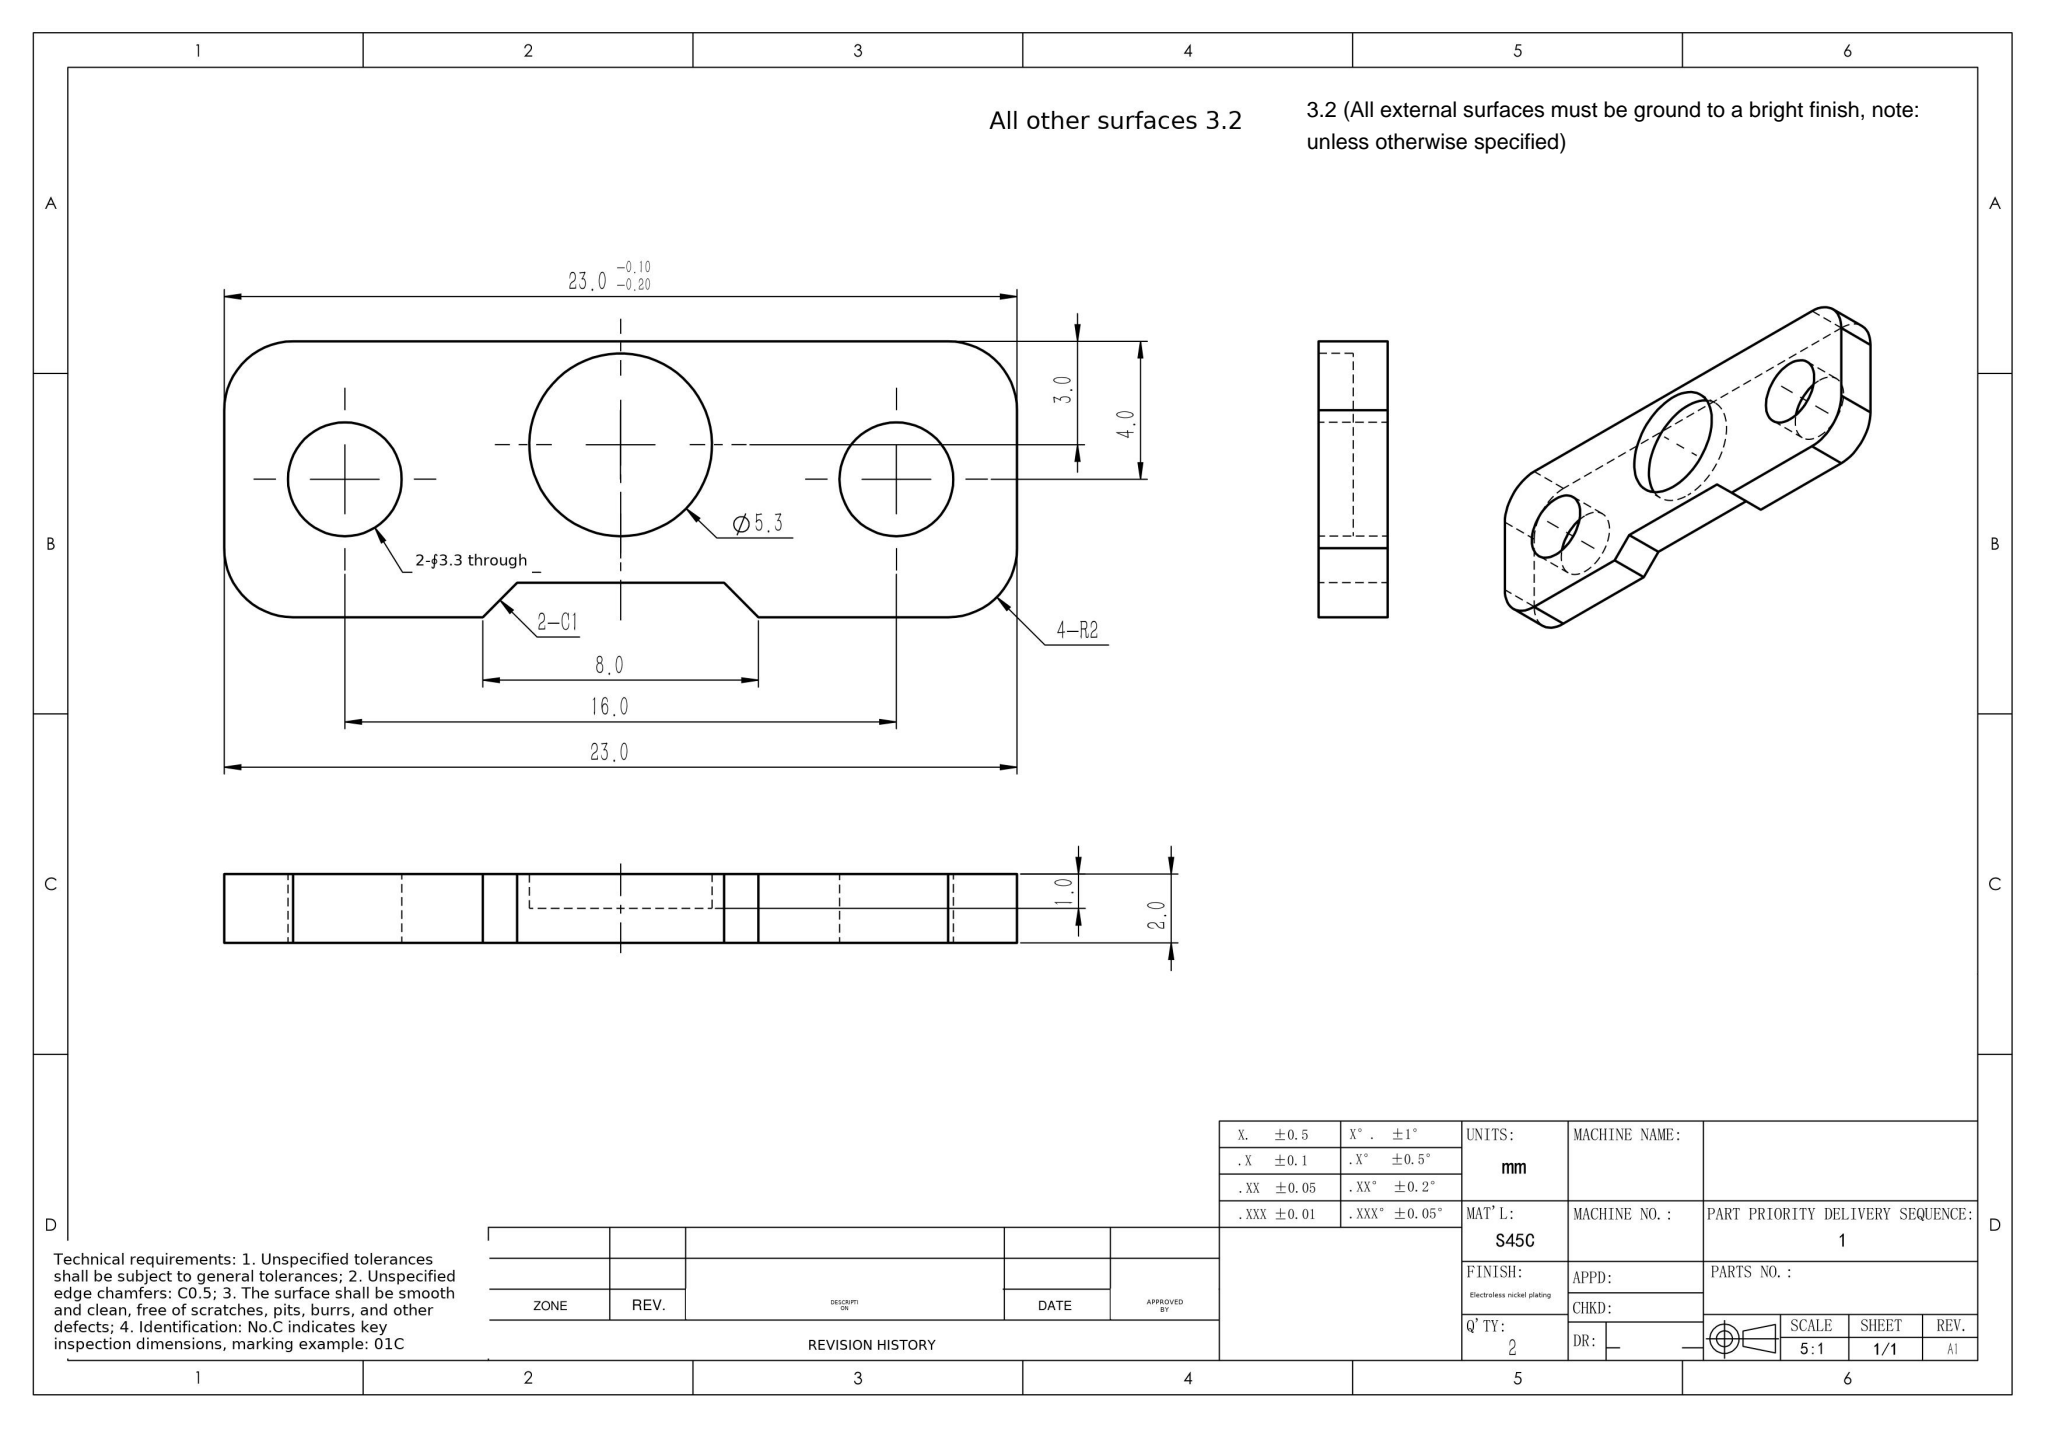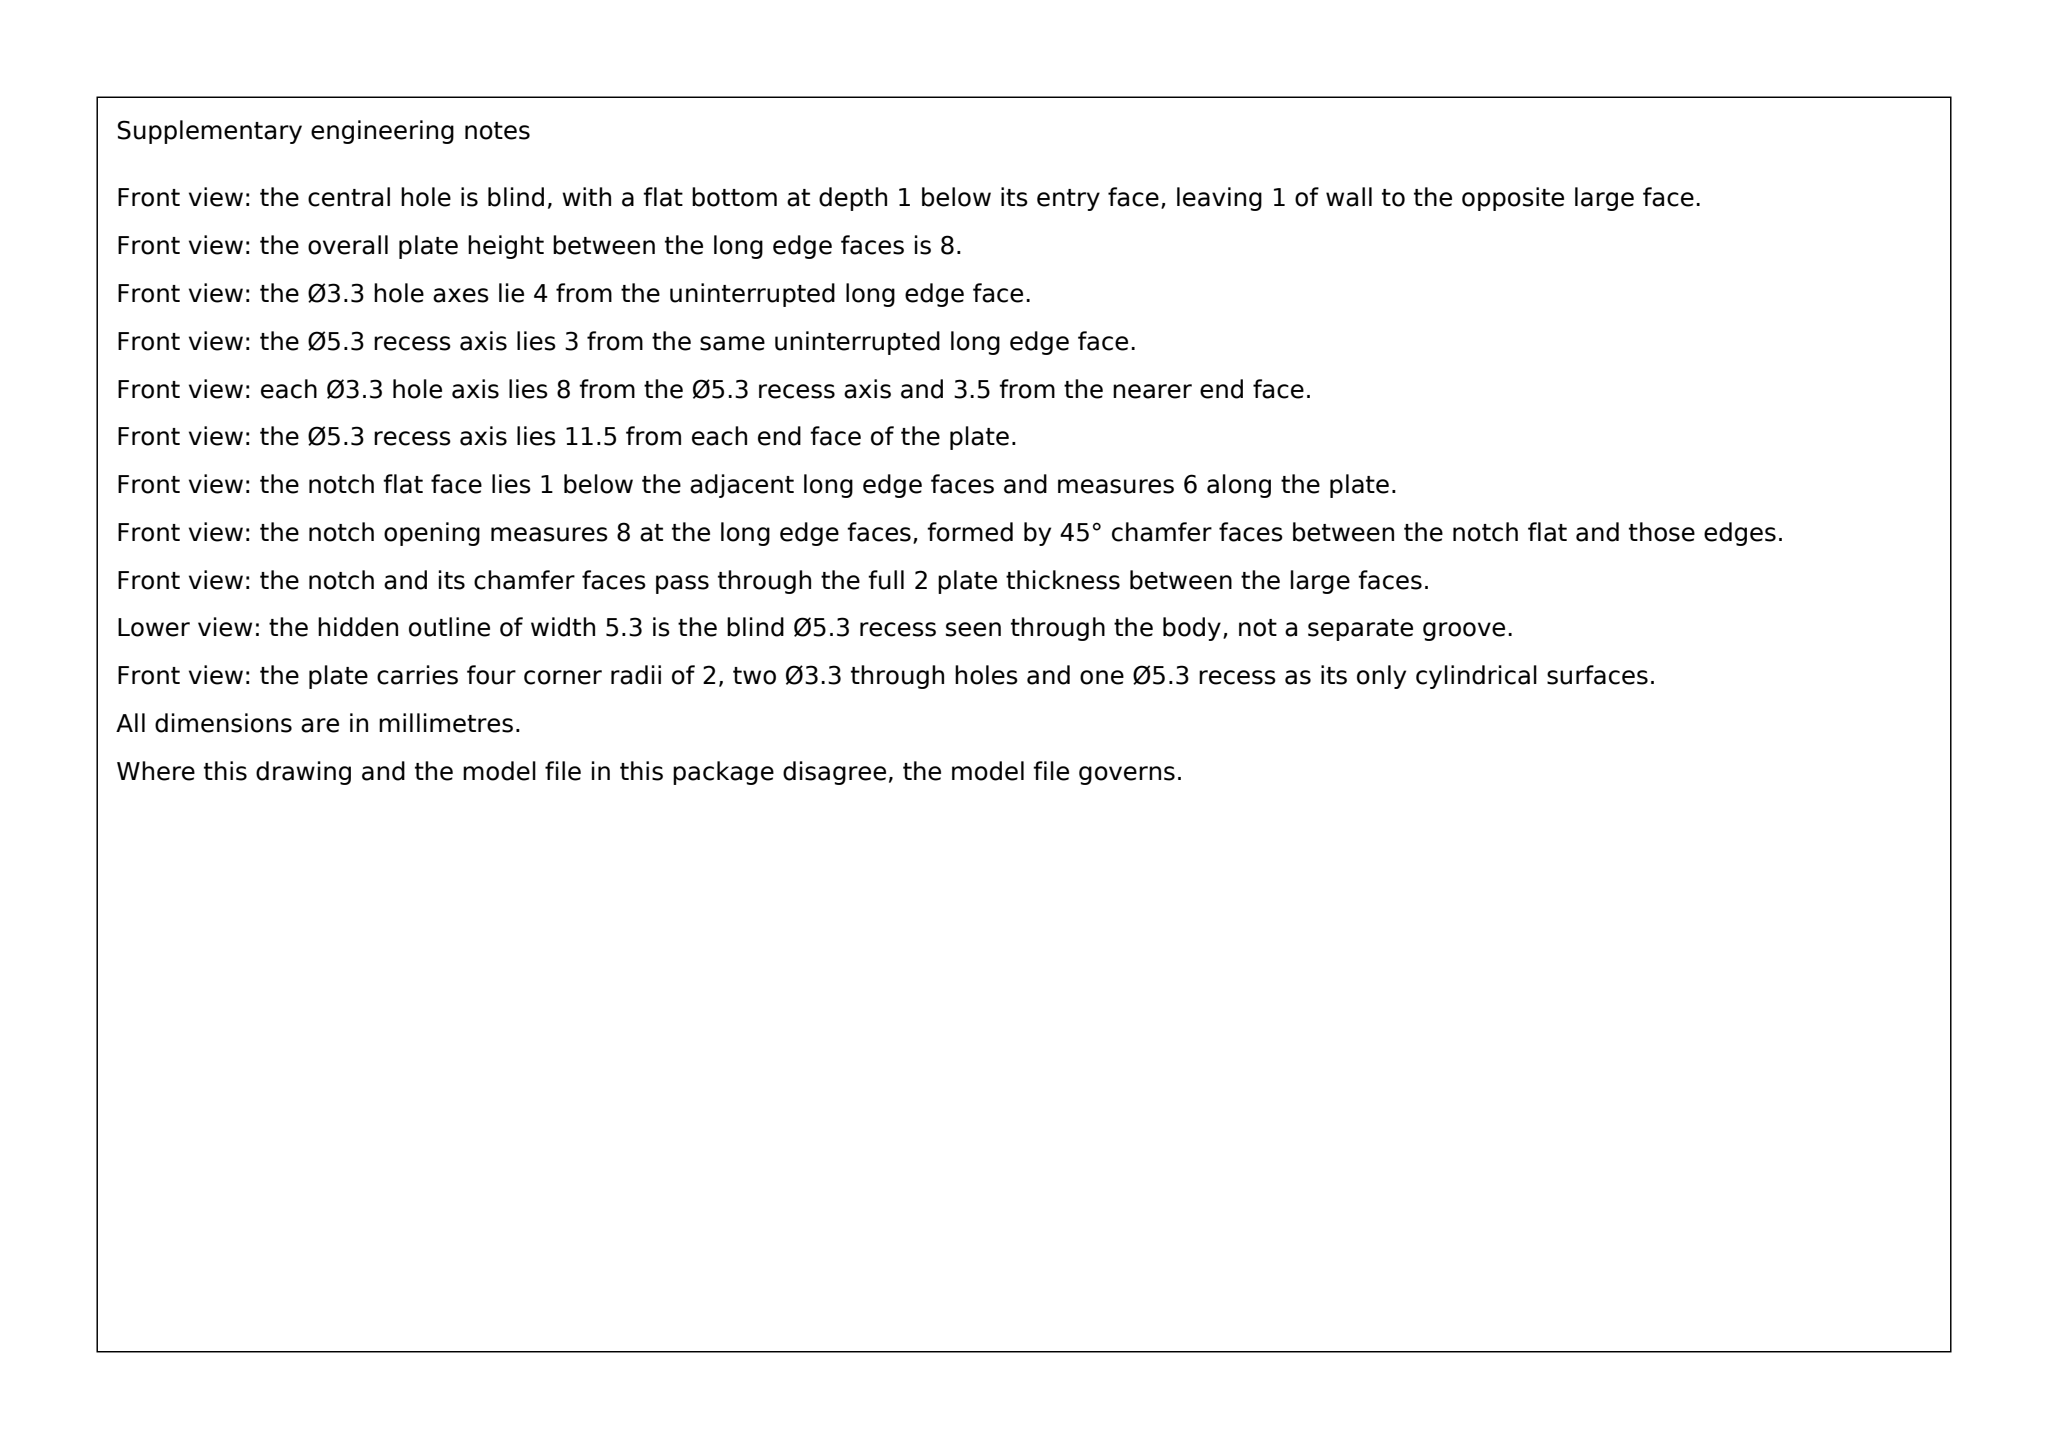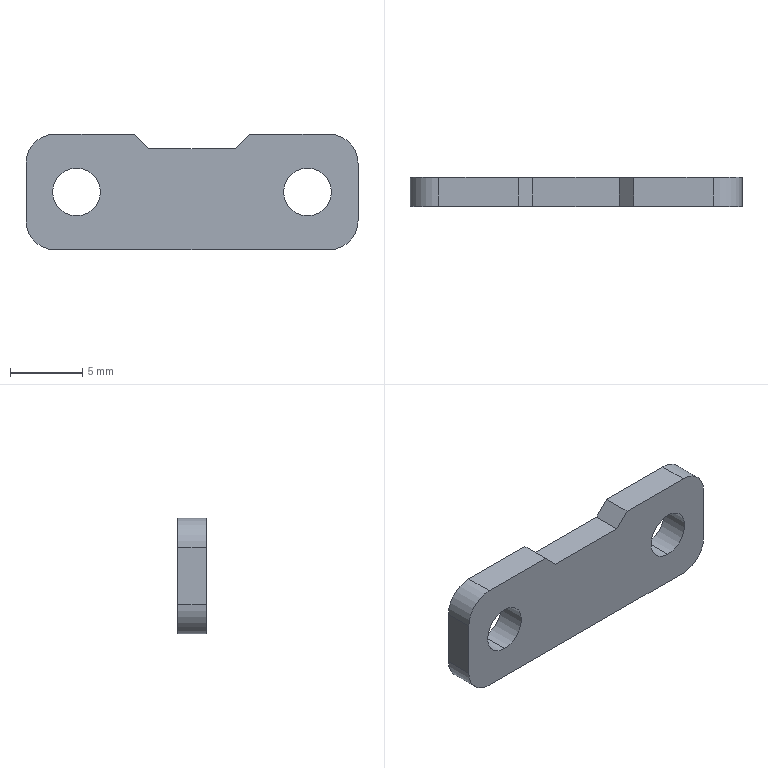Part | SolidWorks | mm | material S45C | 1 solid | 21 faces | box 23 x 2 x 8 mm | volume 291 mm3 | plane 11 | cylinder 10 | commonest cylinder face diameters 3.3 x4 4 x4 5.3 x2
Drawing notes:
Overall height 8.0 from bottom face to top face (plate 23.0 long x 8.0 high x 2.0 thick) | from the solid: bbox_xyz [23.0, 2.0, 8.0]
2X Ø3.3 THRU (2.0 deep), located 3.5 and 19.5 from left end, 4.0 up from bottom edge | from the solid: cylinders dia 3.3, axis y, pos [3.5,null,4.0] and [19.5,null,4.0], length 2.0
Ø5.3 C'BORE 1.0 DEEP both faces, centered 11.5 from left end, 3.0 up from bottom edge | from the solid: cylinders dia 5.3, axis y, pos [11.5,null,3.0], length 1.0, count 2
Overall part width 8.0 across the front view, measured from the back face (Z0 datum). | from the solid: bbox_xyz = [23.0, 2.0, 8.0]
2X Ø3.3 THRU, on hole centerline 4.0 from back face, located 3.5 and 19.5 from left end face (X0 datum). | from the solid: cylinders 3.3 dia, axis y, pos [3.5,null,4.0] and [19.5,null,4.0], length 2.0
Ø5.3 hole, depth 1.0 from each face, center 11.5 from left end face and 3.0 from back face. | from the solid: cylinders 5.3 dia, axis y, pos [11.5,null,3.0], length 1.0, count 2
STEP:
#1=CARTESIAN_POINT('',(8.,2.,-1.65));
#2=VERTEX_POINT('',#1);
#3=CARTESIAN_POINT('',(8.,2.,1.65));
#4=VERTEX_POINT('',#3);
#5=CARTESIAN_POINT('',(8.,2.,0.));
#6=DIRECTION('',(0.,1.,0.));
#7=DIRECTION('',(0.,0.,-1.));
#8=AXIS2_PLACEMENT_3D('',#5,#6,#7);
#9=CIRCLE('',#8,1.65);
#10=EDGE_CURVE('',#2,#4,#9,.T.);
#11=ORIENTED_EDGE('',*,*,#10,.T.);
#12=CARTESIAN_POINT('',(8.,0.,1.65));
#13=VERTEX_POINT('',#12);
#14=CARTESIAN_POINT('',(8.,6.667,1.65));
#15=DIRECTION('',(0.,-1.,0.));
#16=VECTOR('',#15,1000.);
#17=LINE('',#14,#16);
#18=EDGE_CURVE('',#4,#13,#17,.T.);
#19=ORIENTED_EDGE('',*,*,#18,.T.);
#20=CARTESIAN_POINT('',(8.,0.,-1.65));
#21=VERTEX_POINT('',#20);
#22=CARTESIAN_POINT('',(8.,0.,0.));
#23=DIRECTION('',(0.,-1.,0.));
#24=DIRECTION('',(0.,0.,-1.));
#25=AXIS2_PLACEMENT_3D('',#22,#23,#24);
#26=CIRCLE('',#25,1.65);
#27=EDGE_CURVE('',#13,#21,#26,.T.);
#28=ORIENTED_EDGE('',*,*,#27,.T.);
#29=CARTESIAN_POINT('',(8.,6.667,-1.65));
#30=DIRECTION('',(0.,-1.,0.));
#31=VECTOR('',#30,1000.);
#32=LINE('',#29,#31);
#33=EDGE_CURVE('',#2,#21,#32,.T.);
#34=ORIENTED_EDGE('',*,*,#33,.F.);
#35=EDGE_LOOP('',(#11,#19,#28,#34));
#36=FACE_OUTER_BOUND('',#35,.T.);
#37=CARTESIAN_POINT('',(8.,6.667,0.));
#38=DIRECTION('',(0.,-1.,0.));
#39=DIRECTION('',(0.,0.,-1.));
#40=AXIS2_PLACEMENT_3D('',#37,#38,#39);
#41=CYLINDRICAL_SURFACE('',#40,1.65);
#42=ADVANCED_FACE('',(#36),#41,.F.);
#43=CARTESIAN_POINT('',(-8.,2.,-1.65));
#44=VERTEX_POINT('',#43);
#45=CARTESIAN_POINT('',(-8.,2.,1.65));
#46=VERTEX_POINT('',#45);
#47=CARTESIAN_POINT('',(-8.,2.,0.));
#48=DIRECTION('',(0.,1.,0.));
#49=DIRECTION('',(0.,0.,-1.));
#50=AXIS2_PLACEMENT_3D('',#47,#48,#49);
#51=CIRCLE('',#50,1.65);
#52=EDGE_CURVE('',#44,#46,#51,.T.);
#53=ORIENTED_EDGE('',*,*,#52,.T.);
#54=CARTESIAN_POINT('',(-8.,0.,1.65));
#55=VERTEX_POINT('',#54);
#56=CARTESIAN_POINT('',(-8.,6.667,1.65));
#57=DIRECTION('',(0.,-1.,0.));
#58=VECTOR('',#57,1000.);
#59=LINE('',#56,#58);
#60=EDGE_CURVE('',#46,#55,#59,.T.);
#61=ORIENTED_EDGE('',*,*,#60,.T.);
#62=CARTESIAN_POINT('',(-8.,0.,-1.65));
#63=VERTEX_POINT('',#62);
#64=CARTESIAN_POINT('',(-8.,0.,0.));
#65=DIRECTION('',(0.,-1.,0.));
#66=DIRECTION('',(0.,0.,-1.));
#67=AXIS2_PLACEMENT_3D('',#64,#65,#66);
#68=CIRCLE('',#67,1.65);
#69=EDGE_CURVE('',#55,#63,#68,.T.);
#70=ORIENTED_EDGE('',*,*,#69,.T.);
#71=CARTESIAN_POINT('',(-8.,6.667,-1.65));
#72=DIRECTION('',(0.,-1.,0.));
#73=VECTOR('',#72,1000.);
#74=LINE('',#71,#73);
#75=EDGE_CURVE('',#44,#63,#74,.T.);
#76=ORIENTED_EDGE('',*,*,#75,.F.);
#77=EDGE_LOOP('',(#53,#61,#70,#76));
#78=FACE_OUTER_BOUND('',#77,.T.);
#79=CARTESIAN_POINT('',(-8.,6.667,0.));
#80=DIRECTION('',(0.,-1.,0.));
#81=DIRECTION('',(0.,0.,-1.));
#82=AXIS2_PLACEMENT_3D('',#79,#80,#81);
#83=CYLINDRICAL_SURFACE('',#82,1.65);
#84=ADVANCED_FACE('',(#78),#83,.F.);
#85=CARTESIAN_POINT('',(-0.,1.,-3.65));
#86=VERTEX_POINT('',#85);
#87=CARTESIAN_POINT('',(-0.,1.,1.65));
#88=VERTEX_POINT('',#87);
#89=CARTESIAN_POINT('',(-0.,1.,-1.));
#90=DIRECTION('',(0.,1.,0.));
#91=DIRECTION('',(0.,0.,1.));
#92=AXIS2_PLACEMENT_3D('',#89,#90,#91);
#93=CIRCLE('',#92,2.65);
#94=EDGE_CURVE('',#86,#88,#93,.T.);
#95=ORIENTED_EDGE('',*,*,#94,.F.);
#96=CARTESIAN_POINT('',(-0.,2.,-3.65));
#97=VERTEX_POINT('',#96);
#98=CARTESIAN_POINT('',(-0.,1.,-3.65));
#99=DIRECTION('',(0.,1.,0.));
#100=VECTOR('',#99,1000.);
#101=LINE('',#98,#100);
#102=EDGE_CURVE('',#86,#97,#101,.T.);
#103=ORIENTED_EDGE('',*,*,#102,.T.);
#104=CARTESIAN_POINT('',(-0.,2.,1.65));
#105=VERTEX_POINT('',#104);
#106=CARTESIAN_POINT('',(-0.,2.,-1.));
#107=DIRECTION('',(0.,1.,0.));
#108=DIRECTION('',(0.,0.,1.));
#109=AXIS2_PLACEMENT_3D('',#106,#107,#108);
#110=CIRCLE('',#109,2.65);
#111=EDGE_CURVE('',#97,#105,#110,.T.);
#112=ORIENTED_EDGE('',*,*,#111,.T.);
#113=CARTESIAN_POINT('',(-0.,1.,1.65));
#114=DIRECTION('',(0.,1.,0.));
#115=VECTOR('',#114,1000.);
#116=LINE('',#113,#115);
#117=EDGE_CURVE('',#88,#105,#116,.T.);
#118=ORIENTED_EDGE('',*,*,#117,.F.);
#119=EDGE_LOOP('',(#95,#103,#112,#118));
#120=FACE_OUTER_BOUND('',#119,.T.);
#121=CARTESIAN_POINT('',(-0.,1.,-1.));
#122=DIRECTION('',(0.,1.,0.));
#123=DIRECTION('',(0.,0.,1.));
#124=AXIS2_PLACEMENT_3D('',#121,#122,#123);
#125=CYLINDRICAL_SURFACE('',#124,2.65);
#126=ADVANCED_FACE('',(#120),#125,.F.);
#127=CARTESIAN_POINT('',(-4.,2.,4.));
#128=VERTEX_POINT('',#127);
#129=CARTESIAN_POINT('',(-4.,0.,4.));
#130=VERTEX_POINT('',#129);
#131=CARTESIAN_POINT('',(-4.,2.,4.));
#132=DIRECTION('',(0.,-1.,0.));
#133=VECTOR('',#132,1000.);
#134=LINE('',#131,#133);
#135=EDGE_CURVE('',#128,#130,#134,.T.);
#136=ORIENTED_EDGE('',*,*,#135,.F.);
#137=CARTESIAN_POINT('',(-9.5,2.,4.));
#138=VERTEX_POINT('',#137);
#139=CARTESIAN_POINT('',(11.5,2.,4.));
#140=DIRECTION('',(-1.,0.,0.));
#141=VECTOR('',#140,1000.);
#142=LINE('',#139,#141);
#143=EDGE_CURVE('',#128,#138,#142,.T.);
#144=ORIENTED_EDGE('',*,*,#143,.T.);
#145=CARTESIAN_POINT('',(-9.5,0.,4.));
#146=VERTEX_POINT('',#145);
#147=CARTESIAN_POINT('',(-9.5,0.,4.));
#148=DIRECTION('',(0.,-1.,0.));
#149=VECTOR('',#148,1000.);
#150=LINE('',#147,#149);
#151=EDGE_CURVE('',#138,#146,#150,.T.);
#152=ORIENTED_EDGE('',*,*,#151,.T.);
#153=CARTESIAN_POINT('',(-11.5,0.,4.));
#154=DIRECTION('',(1.,0.,0.));
#155=VECTOR('',#154,1000.);
#156=LINE('',#153,#155);
#157=EDGE_CURVE('',#146,#130,#156,.T.);
#158=ORIENTED_EDGE('',*,*,#157,.T.);
#159=EDGE_LOOP('',(#136,#144,#152,#158));
#160=FACE_OUTER_BOUND('',#159,.T.);
#161=CARTESIAN_POINT('',(0.,0.,4.));
#162=DIRECTION('',(0.,0.,1.));
#163=DIRECTION('',(1.,0.,0.));
#164=AXIS2_PLACEMENT_3D('',#161,#162,#163);
#165=PLANE('',#164);
#166=ADVANCED_FACE('',(#160),#165,.T.);
#167=CARTESIAN_POINT('',(-11.5,0.,2.));
#168=VERTEX_POINT('',#167);
#169=CARTESIAN_POINT('',(-11.5,0.,-2.));
#170=VERTEX_POINT('',#169);
#171=CARTESIAN_POINT('',(-11.5,0.,4.));
#172=DIRECTION('',(0.,0.,-1.));
#173=VECTOR('',#172,1000.);
#174=LINE('',#171,#173);
#175=EDGE_CURVE('',#168,#170,#174,.T.);
#176=ORIENTED_EDGE('',*,*,#175,.F.);
#177=CARTESIAN_POINT('',(-11.5,2.,2.));
#178=VERTEX_POINT('',#177);
#179=CARTESIAN_POINT('',(-11.5,2.,2.));
#180=DIRECTION('',(0.,1.,0.));
#181=VECTOR('',#180,1000.);
#182=LINE('',#179,#181);
#183=EDGE_CURVE('',#168,#178,#182,.T.);
#184=ORIENTED_EDGE('',*,*,#183,.T.);
#185=CARTESIAN_POINT('',(-11.5,2.,-2.));
#186=VERTEX_POINT('',#185);
#187=CARTESIAN_POINT('',(-11.5,2.,4.));
#188=DIRECTION('',(0.,0.,-1.));
#189=VECTOR('',#188,1000.);
#190=LINE('',#187,#189);
#191=EDGE_CURVE('',#178,#186,#190,.T.);
#192=ORIENTED_EDGE('',*,*,#191,.T.);
#193=CARTESIAN_POINT('',(-11.5,2.,-2.));
#194=DIRECTION('',(0.,-1.,0.));
#195=VECTOR('',#194,1000.);
#196=LINE('',#193,#195);
#197=EDGE_CURVE('',#186,#170,#196,.T.);
#198=ORIENTED_EDGE('',*,*,#197,.T.);
#199=EDGE_LOOP('',(#176,#184,#192,#198));
#200=FACE_OUTER_BOUND('',#199,.T.);
#201=CARTESIAN_POINT('',(-11.5,2.,4.));
#202=DIRECTION('',(1.,0.,0.));
#203=DIRECTION('',(0.,0.,-1.));
#204=AXIS2_PLACEMENT_3D('',#201,#202,#203);
#205=PLANE('',#204);
#206=ADVANCED_FACE('',(#200),#205,.F.);
#207=CARTESIAN_POINT('',(8.,0.,0.));
#208=DIRECTION('',(0.,-1.,0.));
#209=DIRECTION('',(0.,0.,-1.));
#210=AXIS2_PLACEMENT_3D('',#207,#208,#209);
#211=CIRCLE('',#210,1.65);
#212=EDGE_CURVE('',#21,#13,#211,.T.);
#213=ORIENTED_EDGE('',*,*,#212,.F.);
#214=ORIENTED_EDGE('',*,*,#27,.F.);
#215=EDGE_LOOP('',(#213,#214));
#216=FACE_BOUND('',#215,.T.);
#217=CARTESIAN_POINT('',(-8.,0.,0.));
#218=DIRECTION('',(0.,-1.,0.));
#219=DIRECTION('',(0.,0.,-1.));
#220=AXIS2_PLACEMENT_3D('',#217,#218,#219);
#221=CIRCLE('',#220,1.65);
#222=EDGE_CURVE('',#63,#55,#221,.T.);
#223=ORIENTED_EDGE('',*,*,#222,.F.);
#224=ORIENTED_EDGE('',*,*,#69,.F.);
#225=EDGE_LOOP('',(#223,#224));
#226=FACE_BOUND('',#225,.T.);
#227=CARTESIAN_POINT('',(-3.,0.,3.));
#228=VERTEX_POINT('',#227);
#229=CARTESIAN_POINT('',(3.,0.,3.));
#230=VERTEX_POINT('',#229);
#231=CARTESIAN_POINT('',(-4.,0.,3.));
#232=DIRECTION('',(1.,0.,0.));
#233=VECTOR('',#232,1000.);
#234=LINE('',#231,#233);
#235=EDGE_CURVE('',#228,#230,#234,.T.);
#236=ORIENTED_EDGE('',*,*,#235,.F.);
#237=CARTESIAN_POINT('',(-7.75,0.,7.75));
#238=DIRECTION('',(-0.7071,0.,0.7071));
#239=VECTOR('',#238,1000.);
#240=LINE('',#237,#239);
#241=EDGE_CURVE('',#228,#130,#240,.T.);
#242=ORIENTED_EDGE('',*,*,#241,.T.);
#243=ORIENTED_EDGE('',*,*,#157,.F.);
#244=CARTESIAN_POINT('',(-9.5,0.,2.));
#245=DIRECTION('',(0.,-1.,0.));
#246=DIRECTION('',(0.,0.,1.));
#247=AXIS2_PLACEMENT_3D('',#244,#245,#246);
#248=CIRCLE('',#247,2.);
#249=EDGE_CURVE('',#146,#168,#248,.T.);
#250=ORIENTED_EDGE('',*,*,#249,.T.);
#251=ORIENTED_EDGE('',*,*,#175,.T.);
#252=CARTESIAN_POINT('',(-9.5,0.,-4.));
#253=VERTEX_POINT('',#252);
#254=CARTESIAN_POINT('',(-9.5,0.,-2.));
#255=DIRECTION('',(0.,-1.,0.));
#256=DIRECTION('',(0.,0.,1.));
#257=AXIS2_PLACEMENT_3D('',#254,#255,#256);
#258=CIRCLE('',#257,2.);
#259=EDGE_CURVE('',#170,#253,#258,.T.);
#260=ORIENTED_EDGE('',*,*,#259,.T.);
#261=CARTESIAN_POINT('',(9.5,0.,-4.));
#262=VERTEX_POINT('',#261);
#263=CARTESIAN_POINT('',(-11.5,0.,-4.));
#264=DIRECTION('',(1.,0.,0.));
#265=VECTOR('',#264,1000.);
#266=LINE('',#263,#265);
#267=EDGE_CURVE('',#253,#262,#266,.T.);
#268=ORIENTED_EDGE('',*,*,#267,.T.);
#269=CARTESIAN_POINT('',(11.5,0.,-2.));
#270=VERTEX_POINT('',#269);
#271=CARTESIAN_POINT('',(9.5,0.,-2.));
#272=DIRECTION('',(0.,-1.,0.));
#273=DIRECTION('',(0.,0.,1.));
#274=AXIS2_PLACEMENT_3D('',#271,#272,#273);
#275=CIRCLE('',#274,2.);
#276=EDGE_CURVE('',#262,#270,#275,.T.);
#277=ORIENTED_EDGE('',*,*,#276,.T.);
#278=CARTESIAN_POINT('',(11.5,0.,2.));
#279=VERTEX_POINT('',#278);
#280=CARTESIAN_POINT('',(11.5,0.,4.));
#281=DIRECTION('',(0.,0.,-1.));
#282=VECTOR('',#281,1000.);
#283=LINE('',#280,#282);
#284=EDGE_CURVE('',#279,#270,#283,.T.);
#285=ORIENTED_EDGE('',*,*,#284,.F.);
#286=CARTESIAN_POINT('',(9.5,0.,4.));
#287=VERTEX_POINT('',#286);
#288=CARTESIAN_POINT('',(9.5,0.,2.));
#289=DIRECTION('',(0.,-1.,0.));
#290=DIRECTION('',(0.,0.,1.));
#291=AXIS2_PLACEMENT_3D('',#288,#289,#290);
#292=CIRCLE('',#291,2.);
#293=EDGE_CURVE('',#279,#287,#292,.T.);
#294=ORIENTED_EDGE('',*,*,#293,.T.);
#295=CARTESIAN_POINT('',(4.,0.,4.));
#296=VERTEX_POINT('',#295);
#297=CARTESIAN_POINT('',(-11.5,0.,4.));
#298=DIRECTION('',(1.,0.,0.));
#299=VECTOR('',#298,1000.);
#300=LINE('',#297,#299);
#301=EDGE_CURVE('',#296,#287,#300,.T.);
#302=ORIENTED_EDGE('',*,*,#301,.F.);
#303=CARTESIAN_POINT('',(-3.75,0.,-3.75));
#304=DIRECTION('',(-0.7071,0.,-0.7071));
#305=VECTOR('',#304,1000.);
#306=LINE('',#303,#305);
#307=EDGE_CURVE('',#296,#230,#306,.T.);
#308=ORIENTED_EDGE('',*,*,#307,.T.);
#309=EDGE_LOOP('',(#236,#242,#243,#250,#251,#260,#268,#277,#285,#294,#302,#308));
#310=FACE_OUTER_BOUND('',#309,.T.);
#311=CARTESIAN_POINT('',(-11.5,0.,4.));
#312=DIRECTION('',(0.,1.,0.));
#313=DIRECTION('',(0.,0.,1.));
#314=AXIS2_PLACEMENT_3D('',#311,#312,#313);
#315=PLANE('',#314);
#316=ADVANCED_FACE('',(#216,#226,#310),#315,.F.);
#317=CARTESIAN_POINT('',(11.5,2.,2.));
#318=VERTEX_POINT('',#317);
#319=CARTESIAN_POINT('',(11.5,2.,-2.));
#320=VERTEX_POINT('',#319);
#321=CARTESIAN_POINT('',(11.5,2.,4.));
#322=DIRECTION('',(0.,0.,-1.));
#323=VECTOR('',#322,1000.);
#324=LINE('',#321,#323);
#325=EDGE_CURVE('',#318,#320,#324,.T.);
#326=ORIENTED_EDGE('',*,*,#325,.F.);
#327=CARTESIAN_POINT('',(11.5,0.,2.));
#328=DIRECTION('',(0.,-1.,0.));
#329=VECTOR('',#328,1000.);
#330=LINE('',#327,#329);
#331=EDGE_CURVE('',#318,#279,#330,.T.);
#332=ORIENTED_EDGE('',*,*,#331,.T.);
#333=ORIENTED_EDGE('',*,*,#284,.T.);
#334=CARTESIAN_POINT('',(11.5,0.,-2.));
#335=DIRECTION('',(0.,1.,0.));
#336=VECTOR('',#335,1000.);
#337=LINE('',#334,#336);
#338=EDGE_CURVE('',#270,#320,#337,.T.);
#339=ORIENTED_EDGE('',*,*,#338,.T.);
#340=EDGE_LOOP('',(#326,#332,#333,#339));
#341=FACE_OUTER_BOUND('',#340,.T.);
#342=CARTESIAN_POINT('',(11.5,0.,4.));
#343=DIRECTION('',(-1.,0.,0.));
#344=DIRECTION('',(0.,0.,1.));
#345=AXIS2_PLACEMENT_3D('',#342,#343,#344);
#346=PLANE('',#345);
#347=ADVANCED_FACE('',(#341),#346,.F.);
#348=ORIENTED_EDGE('',*,*,#10,.F.);
#349=CARTESIAN_POINT('',(8.,2.,0.));
#350=DIRECTION('',(0.,1.,0.));
#351=DIRECTION('',(0.,0.,-1.));
#352=AXIS2_PLACEMENT_3D('',#349,#350,#351);
#353=CIRCLE('',#352,1.65);
#354=EDGE_CURVE('',#4,#2,#353,.T.);
#355=ORIENTED_EDGE('',*,*,#354,.F.);
#356=EDGE_LOOP('',(#348,#355));
#357=FACE_BOUND('',#356,.T.);
#358=ORIENTED_EDGE('',*,*,#52,.F.);
#359=CARTESIAN_POINT('',(-8.,2.,0.));
#360=DIRECTION('',(0.,1.,0.));
#361=DIRECTION('',(0.,0.,-1.));
#362=AXIS2_PLACEMENT_3D('',#359,#360,#361);
#363=CIRCLE('',#362,1.65);
#364=EDGE_CURVE('',#46,#44,#363,.T.);
#365=ORIENTED_EDGE('',*,*,#364,.F.);
#366=EDGE_LOOP('',(#358,#365));
#367=FACE_BOUND('',#366,.T.);
#368=CARTESIAN_POINT('',(-0.,2.,-1.));
#369=DIRECTION('',(0.,1.,0.));
#370=DIRECTION('',(0.,0.,1.));
#371=AXIS2_PLACEMENT_3D('',#368,#369,#370);
#372=CIRCLE('',#371,2.65);
#373=EDGE_CURVE('',#105,#97,#372,.T.);
#374=ORIENTED_EDGE('',*,*,#373,.F.);
#375=ORIENTED_EDGE('',*,*,#111,.F.);
#376=EDGE_LOOP('',(#374,#375));
#377=FACE_BOUND('',#376,.T.);
#378=ORIENTED_EDGE('',*,*,#143,.F.);
#379=CARTESIAN_POINT('',(-3.,2.,3.));
#380=VERTEX_POINT('',#379);
#381=CARTESIAN_POINT('',(3.75,2.,-3.75));
#382=DIRECTION('',(0.7071,0.,-0.7071));
#383=VECTOR('',#382,1000.);
#384=LINE('',#381,#383);
#385=EDGE_CURVE('',#128,#380,#384,.T.);
#386=ORIENTED_EDGE('',*,*,#385,.T.);
#387=CARTESIAN_POINT('',(3.,2.,3.));
#388=VERTEX_POINT('',#387);
#389=CARTESIAN_POINT('',(-4.,2.,3.));
#390=DIRECTION('',(1.,0.,0.));
#391=VECTOR('',#390,1000.);
#392=LINE('',#389,#391);
#393=EDGE_CURVE('',#380,#388,#392,.T.);
#394=ORIENTED_EDGE('',*,*,#393,.T.);
#395=CARTESIAN_POINT('',(4.,2.,4.));
#396=VERTEX_POINT('',#395);
#397=CARTESIAN_POINT('',(7.75,2.,7.75));
#398=DIRECTION('',(0.7071,0.,0.7071));
#399=VECTOR('',#398,1000.);
#400=LINE('',#397,#399);
#401=EDGE_CURVE('',#388,#396,#400,.T.);
#402=ORIENTED_EDGE('',*,*,#401,.T.);
#403=CARTESIAN_POINT('',(9.5,2.,4.));
#404=VERTEX_POINT('',#403);
#405=CARTESIAN_POINT('',(11.5,2.,4.));
#406=DIRECTION('',(-1.,0.,0.));
#407=VECTOR('',#406,1000.);
#408=LINE('',#405,#407);
#409=EDGE_CURVE('',#404,#396,#408,.T.);
#410=ORIENTED_EDGE('',*,*,#409,.F.);
#411=CARTESIAN_POINT('',(9.5,2.,2.));
#412=DIRECTION('',(0.,1.,0.));
#413=DIRECTION('',(0.,0.,-1.));
#414=AXIS2_PLACEMENT_3D('',#411,#412,#413);
#415=CIRCLE('',#414,2.);
#416=EDGE_CURVE('',#404,#318,#415,.T.);
#417=ORIENTED_EDGE('',*,*,#416,.T.);
#418=ORIENTED_EDGE('',*,*,#325,.T.);
#419=CARTESIAN_POINT('',(9.5,2.,-4.));
#420=VERTEX_POINT('',#419);
#421=CARTESIAN_POINT('',(9.5,2.,-2.));
#422=DIRECTION('',(0.,1.,0.));
#423=DIRECTION('',(0.,0.,-1.));
#424=AXIS2_PLACEMENT_3D('',#421,#422,#423);
#425=CIRCLE('',#424,2.);
#426=EDGE_CURVE('',#320,#420,#425,.T.);
#427=ORIENTED_EDGE('',*,*,#426,.T.);
#428=CARTESIAN_POINT('',(-9.5,2.,-4.));
#429=VERTEX_POINT('',#428);
#430=CARTESIAN_POINT('',(11.5,2.,-4.));
#431=DIRECTION('',(-1.,0.,0.));
#432=VECTOR('',#431,1000.);
#433=LINE('',#430,#432);
#434=EDGE_CURVE('',#420,#429,#433,.T.);
#435=ORIENTED_EDGE('',*,*,#434,.T.);
#436=CARTESIAN_POINT('',(-9.5,2.,-2.));
#437=DIRECTION('',(0.,1.,0.));
#438=DIRECTION('',(0.,0.,-1.));
#439=AXIS2_PLACEMENT_3D('',#436,#437,#438);
#440=CIRCLE('',#439,2.);
#441=EDGE_CURVE('',#429,#186,#440,.T.);
#442=ORIENTED_EDGE('',*,*,#441,.T.);
#443=ORIENTED_EDGE('',*,*,#191,.F.);
#444=CARTESIAN_POINT('',(-9.5,2.,2.));
#445=DIRECTION('',(0.,1.,0.));
#446=DIRECTION('',(0.,0.,-1.));
#447=AXIS2_PLACEMENT_3D('',#444,#445,#446);
#448=CIRCLE('',#447,2.);
#449=EDGE_CURVE('',#178,#138,#448,.T.);
#450=ORIENTED_EDGE('',*,*,#449,.T.);
#451=EDGE_LOOP('',(#378,#386,#394,#402,#410,#417,#418,#427,#435,#442,#443,#450));
#452=FACE_OUTER_BOUND('',#451,.T.);
#453=CARTESIAN_POINT('',(11.5,2.,4.));
#454=DIRECTION('',(0.,-1.,0.));
#455=DIRECTION('',(0.,0.,-1.));
#456=AXIS2_PLACEMENT_3D('',#453,#454,#455);
#457=PLANE('',#456);
#458=ADVANCED_FACE('',(#357,#367,#377,#452),#457,.F.);
#459=CARTESIAN_POINT('',(4.,2.,4.));
#460=DIRECTION('',(0.,-1.,0.));
#461=VECTOR('',#460,1000.);
#462=LINE('',#459,#461);
#463=EDGE_CURVE('',#396,#296,#462,.T.);
#464=ORIENTED_EDGE('',*,*,#463,.T.);
#465=ORIENTED_EDGE('',*,*,#301,.T.);
#466=CARTESIAN_POINT('',(9.5,2.,4.));
#467=DIRECTION('',(0.,1.,0.));
#468=VECTOR('',#467,1000.);
#469=LINE('',#466,#468);
#470=EDGE_CURVE('',#287,#404,#469,.T.);
#471=ORIENTED_EDGE('',*,*,#470,.T.);
#472=ORIENTED_EDGE('',*,*,#409,.T.);
#473=EDGE_LOOP('',(#464,#465,#471,#472));
#474=FACE_OUTER_BOUND('',#473,.T.);
#475=CARTESIAN_POINT('',(0.,0.,4.));
#476=DIRECTION('',(0.,0.,1.));
#477=DIRECTION('',(1.,0.,0.));
#478=AXIS2_PLACEMENT_3D('',#475,#476,#477);
#479=PLANE('',#478);
#480=ADVANCED_FACE('',(#474),#479,.T.);
#481=ORIENTED_EDGE('',*,*,#267,.F.);
#482=CARTESIAN_POINT('',(-9.5,0.,-4.));
#483=DIRECTION('',(0.,1.,0.));
#484=VECTOR('',#483,1000.);
#485=LINE('',#482,#484);
#486=EDGE_CURVE('',#253,#429,#485,.T.);
#487=ORIENTED_EDGE('',*,*,#486,.T.);
#488=ORIENTED_EDGE('',*,*,#434,.F.);
#489=CARTESIAN_POINT('',(9.5,0.,-4.));
#490=DIRECTION('',(0.,-1.,0.));
#491=VECTOR('',#490,1000.);
#492=LINE('',#489,#491);
#493=EDGE_CURVE('',#420,#262,#492,.T.);
#494=ORIENTED_EDGE('',*,*,#493,.T.);
#495=EDGE_LOOP('',(#481,#487,#488,#494));
#496=FACE_OUTER_BOUND('',#495,.T.);
#497=CARTESIAN_POINT('',(0.,0.,-4.));
#498=DIRECTION('',(0.,0.,1.));
#499=DIRECTION('',(1.,0.,0.));
#500=AXIS2_PLACEMENT_3D('',#497,#498,#499);
#501=PLANE('',#500);
#502=ADVANCED_FACE('',(#496),#501,.F.);
#503=ORIENTED_EDGE('',*,*,#449,.F.);
#504=ORIENTED_EDGE('',*,*,#183,.F.);
#505=ORIENTED_EDGE('',*,*,#249,.F.);
#506=ORIENTED_EDGE('',*,*,#151,.F.);
#507=EDGE_LOOP('',(#503,#504,#505,#506));
#508=FACE_OUTER_BOUND('',#507,.T.);
#509=CARTESIAN_POINT('',(-9.5,0.,2.));
#510=DIRECTION('',(0.,1.,0.));
#511=DIRECTION('',(0.,0.,1.));
#512=AXIS2_PLACEMENT_3D('',#509,#510,#511);
#513=CYLINDRICAL_SURFACE('',#512,2.);
#514=ADVANCED_FACE('',(#508),#513,.T.);
#515=ORIENTED_EDGE('',*,*,#441,.F.);
#516=ORIENTED_EDGE('',*,*,#486,.F.);
#517=ORIENTED_EDGE('',*,*,#259,.F.);
#518=ORIENTED_EDGE('',*,*,#197,.F.);
#519=EDGE_LOOP('',(#515,#516,#517,#518));
#520=FACE_OUTER_BOUND('',#519,.T.);
#521=CARTESIAN_POINT('',(-9.5,2.,-2.));
#522=DIRECTION('',(0.,-1.,0.));
#523=DIRECTION('',(0.,0.,-1.));
#524=AXIS2_PLACEMENT_3D('',#521,#522,#523);
#525=CYLINDRICAL_SURFACE('',#524,2.);
#526=ADVANCED_FACE('',(#520),#525,.T.);
#527=ORIENTED_EDGE('',*,*,#293,.F.);
#528=ORIENTED_EDGE('',*,*,#331,.F.);
#529=ORIENTED_EDGE('',*,*,#416,.F.);
#530=ORIENTED_EDGE('',*,*,#470,.F.);
#531=EDGE_LOOP('',(#527,#528,#529,#530));
#532=FACE_OUTER_BOUND('',#531,.T.);
#533=CARTESIAN_POINT('',(9.5,0.,2.));
#534=DIRECTION('',(0.,-1.,0.));
#535=DIRECTION('',(0.,0.,-1.));
#536=AXIS2_PLACEMENT_3D('',#533,#534,#535);
#537=CYLINDRICAL_SURFACE('',#536,2.);
#538=ADVANCED_FACE('',(#532),#537,.T.);
#539=ORIENTED_EDGE('',*,*,#276,.F.);
#540=ORIENTED_EDGE('',*,*,#493,.F.);
#541=ORIENTED_EDGE('',*,*,#426,.F.);
#542=ORIENTED_EDGE('',*,*,#338,.F.);
#543=EDGE_LOOP('',(#539,#540,#541,#542));
#544=FACE_OUTER_BOUND('',#543,.T.);
#545=CARTESIAN_POINT('',(9.5,0.,-2.));
#546=DIRECTION('',(0.,1.,0.));
#547=DIRECTION('',(0.,0.,1.));
#548=AXIS2_PLACEMENT_3D('',#545,#546,#547);
#549=CYLINDRICAL_SURFACE('',#548,2.);
#550=ADVANCED_FACE('',(#544),#549,.T.);
#551=ORIENTED_EDGE('',*,*,#235,.T.);
#552=CARTESIAN_POINT('',(3.,2.,3.));
#553=DIRECTION('',(0.,1.,0.));
#554=VECTOR('',#553,1000.);
#555=LINE('',#552,#554);
#556=EDGE_CURVE('',#230,#388,#555,.T.);
#557=ORIENTED_EDGE('',*,*,#556,.T.);
#558=ORIENTED_EDGE('',*,*,#393,.F.);
#559=CARTESIAN_POINT('',(-3.,0.,3.));
#560=DIRECTION('',(0.,-1.,0.));
#561=VECTOR('',#560,1000.);
#562=LINE('',#559,#561);
#563=EDGE_CURVE('',#380,#228,#562,.T.);
#564=ORIENTED_EDGE('',*,*,#563,.T.);
#565=EDGE_LOOP('',(#551,#557,#558,#564));
#566=FACE_OUTER_BOUND('',#565,.T.);
#567=CARTESIAN_POINT('',(-4.,2.,3.));
#568=DIRECTION('',(0.,0.,-1.));
#569=DIRECTION('',(-1.,0.,-0.));
#570=AXIS2_PLACEMENT_3D('',#567,#568,#569);
#571=PLANE('',#570);
#572=ADVANCED_FACE('',(#566),#571,.F.);
#573=ORIENTED_EDGE('',*,*,#401,.F.);
#574=ORIENTED_EDGE('',*,*,#556,.F.);
#575=ORIENTED_EDGE('',*,*,#307,.F.);
#576=ORIENTED_EDGE('',*,*,#463,.F.);
#577=EDGE_LOOP('',(#573,#574,#575,#576));
#578=FACE_OUTER_BOUND('',#577,.T.);
#579=CARTESIAN_POINT('',(4.,2.,4.));
#580=DIRECTION('',(-0.7071,0.,0.7071));
#581=DIRECTION('',(0.,1.,0.));
#582=AXIS2_PLACEMENT_3D('',#579,#580,#581);
#583=PLANE('',#582);
#584=ADVANCED_FACE('',(#578),#583,.T.);
#585=ORIENTED_EDGE('',*,*,#385,.F.);
#586=ORIENTED_EDGE('',*,*,#135,.T.);
#587=ORIENTED_EDGE('',*,*,#241,.F.);
#588=ORIENTED_EDGE('',*,*,#563,.F.);
#589=EDGE_LOOP('',(#585,#586,#587,#588));
#590=FACE_OUTER_BOUND('',#589,.T.);
#591=CARTESIAN_POINT('',(-3.,2.,3.));
#592=DIRECTION('',(0.7071,0.,0.7071));
#593=DIRECTION('',(0.,1.,0.));
#594=AXIS2_PLACEMENT_3D('',#591,#592,#593);
#595=PLANE('',#594);
#596=ADVANCED_FACE('',(#590),#595,.T.);
#597=ORIENTED_EDGE('',*,*,#102,.F.);
#598=CARTESIAN_POINT('',(-0.,1.,-1.));
#599=DIRECTION('',(0.,1.,0.));
#600=DIRECTION('',(0.,0.,1.));
#601=AXIS2_PLACEMENT_3D('',#598,#599,#600);
#602=CIRCLE('',#601,2.65);
#603=EDGE_CURVE('',#88,#86,#602,.T.);
#604=ORIENTED_EDGE('',*,*,#603,.F.);
#605=ORIENTED_EDGE('',*,*,#117,.T.);
#606=ORIENTED_EDGE('',*,*,#373,.T.);
#607=EDGE_LOOP('',(#597,#604,#605,#606));
#608=FACE_OUTER_BOUND('',#607,.T.);
#609=CARTESIAN_POINT('',(-0.,1.,-1.));
#610=DIRECTION('',(0.,1.,0.));
#611=DIRECTION('',(0.,0.,1.));
#612=AXIS2_PLACEMENT_3D('',#609,#610,#611);
#613=CYLINDRICAL_SURFACE('',#612,2.65);
#614=ADVANCED_FACE('',(#608),#613,.F.);
#615=ORIENTED_EDGE('',*,*,#603,.T.);
#616=ORIENTED_EDGE('',*,*,#94,.T.);
#617=EDGE_LOOP('',(#615,#616));
#618=FACE_OUTER_BOUND('',#617,.T.);
#619=CARTESIAN_POINT('',(-0.,1.,-1.));
#620=DIRECTION('',(0.,1.,0.));
#621=DIRECTION('',(0.,0.,1.));
#622=AXIS2_PLACEMENT_3D('',#619,#620,#621);
#623=PLANE('',#622);
#624=ADVANCED_FACE('',(#618),#623,.T.);
#625=ORIENTED_EDGE('',*,*,#60,.F.);
#626=ORIENTED_EDGE('',*,*,#364,.T.);
#627=ORIENTED_EDGE('',*,*,#75,.T.);
#628=ORIENTED_EDGE('',*,*,#222,.T.);
#629=EDGE_LOOP('',(#625,#626,#627,#628));
#630=FACE_OUTER_BOUND('',#629,.T.);
#631=CARTESIAN_POINT('',(-8.,6.667,0.));
#632=DIRECTION('',(0.,-1.,0.));
#633=DIRECTION('',(0.,0.,-1.));
#634=AXIS2_PLACEMENT_3D('',#631,#632,#633);
#635=CYLINDRICAL_SURFACE('',#634,1.65);
#636=ADVANCED_FACE('',(#630),#635,.F.);
#637=ORIENTED_EDGE('',*,*,#18,.F.);
#638=ORIENTED_EDGE('',*,*,#354,.T.);
#639=ORIENTED_EDGE('',*,*,#33,.T.);
#640=ORIENTED_EDGE('',*,*,#212,.T.);
#641=EDGE_LOOP('',(#637,#638,#639,#640));
#642=FACE_OUTER_BOUND('',#641,.T.);
#643=CARTESIAN_POINT('',(8.,6.667,0.));
#644=DIRECTION('',(0.,-1.,0.));
#645=DIRECTION('',(0.,0.,-1.));
#646=AXIS2_PLACEMENT_3D('',#643,#644,#645);
#647=CYLINDRICAL_SURFACE('',#646,1.65);
#648=ADVANCED_FACE('',(#642),#647,.F.);
#649=CLOSED_SHELL('',(#42,#84,#126,#166,#206,#316,#347,#458,#480,#502,#514,#526,#538,#550,#572,#584,#596,#614,#624,#636,#648));
#650=MANIFOLD_SOLID_BREP('',#649);
#651=CARTESIAN_POINT('',(0.,0.,0.));
#652=DIRECTION('',(0.,0.,1.));
#653=DIRECTION('',(1.,0.,0.));
#654=AXIS2_PLACEMENT_3D('',#651,#652,#653);
#655=(LENGTH_UNIT()NAMED_UNIT(*)SI_UNIT(.MILLI.,.METRE.));
#656=UNCERTAINTY_MEASURE_WITH_UNIT(LENGTH_MEASURE(0.00001),#655,'','');
#657=(NAMED_UNIT(*)PLANE_ANGLE_UNIT()SI_UNIT($,.RADIAN.));
#658=(NAMED_UNIT(*)SI_UNIT($,.STERADIAN.)SOLID_ANGLE_UNIT());
#659=(GEOMETRIC_REPRESENTATION_CONTEXT(3)GLOBAL_UNCERTAINTY_ASSIGNED_CONTEXT((#656))GLOBAL_UNIT_ASSIGNED_CONTEXT((#655,#657,#658))REPRESENTATION_CONTEXT('',''));
#660=ADVANCED_BREP_SHAPE_REPRESENTATION('',(#650,#654),#659);